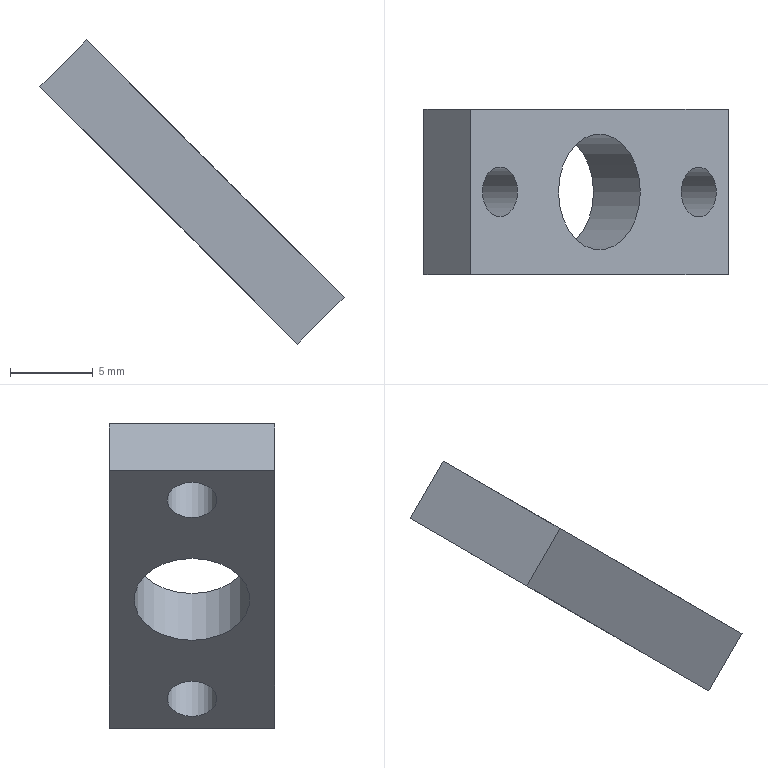Component | NX | INCLINED_FRAME_TOP_PLATE_3 | 1 solid | 9 faces | volume 670 mm3 | plane 6 | cylinder 3 | commonest cylinder face diameters 3 x2 7 x1